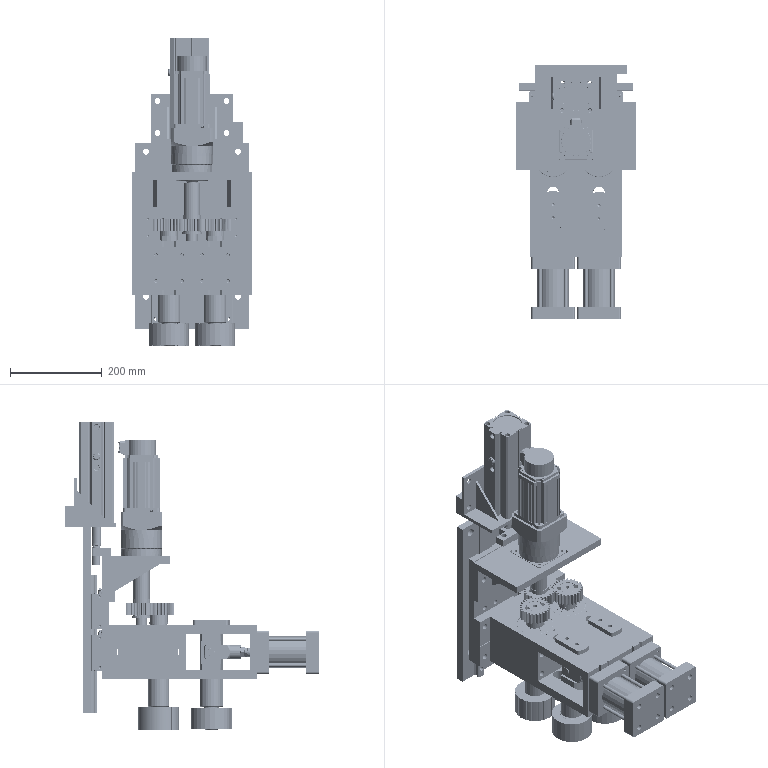Assembly | SolidWorks | mm | 89 component files | 297 solids | 8207 faces | box 260 x 553 x 669.11 mm | volume 14748799 mm3 | plane 3298 | cylinder 2702 | sphere 920 | cone 754 | torus 297 | spline 236 | commonest cylinder face diameters 0.4 x322 10.8 x192 39.85 x160 37.15 x160 4.6 x88 5 x78 67.5 x75 56.25 x75
Bill of materials:
NewCurveBender6203Bearing-DoubleWheel | 1 |  | Thick annular ring with a plain central bore and rounded outer and inner edges.
NewCurveBender6205RZBearing-DoubleWheel | 4 |  | Short, thick annular ring with a plain through bore, a cylindrical outer face and small edge rounds. Each face shows concentric steps or grooves between the inner and outer rims, so the ring looks like it is built from separate inner and outer rings with a recessed band between them.
NewCurveBender6208RSBearing-DoubleWheel | 4 |  | Plain flat annular ring (washer- or spacer-like) with a central through bore. The ring is wide and the part is thin compared with its diameter. The edges are slightly rounded or chamfered.
NewTypeCurveBender34320001-DoubleWheel | 4 |  | Angled fitting: cylindrical shank with chamfered end, a hex collar, a domed body, and an angled branch with a second hex flat and a tapered nozzle with a small orifice.
NewTypeCurveBender920018A1-DoubleWheel | 8 |  | Flat rectangular plate with chamfered corners, a central U-shaped notch with rounded side reliefs, two small through holes and one larger round through hole.
NewTypeCurveBenderDoubleWheel | 4 |  | Cylindrical cap-like body with a thin flange at the base and a chamfered top edge to a flat top face.
NewTypeCurveBenderHG20-DoubleWheel | 16 |  | Round-head pin or screw-like part with a cross-shaped recess in a low domed head and a plain cylindrical shank with chamfered tip.
NewTypeCurveBenderHGH20CAZ0C-DoubleWheel | 4 |  | Rectangular block with a U-channel end profile (chamfered corners, rounded side reliefs), a large cone-bottomed hole and two smaller holes on the end face, cone-bottomed holes on the side faces, and shallow lengthwise grooves and steps.
NewCurveBenderHGW20GuideRail210Long-DoubleWheel | 2 |  | Long straight bar with a constant profile (chamfered top corners, angled side recesses, rounded side grooves near the base) and a row of evenly spaced counterbored through holes along its length.
NewCurveBenderLowerRebarWheelAxis-DoubleWheel | 2 | 45 | Stepped cylindrical shaft with two opposite slots at one end, a small conical centre hole in that end face, circumferential grooves, a larger diameter collar section and a smaller end stub.
NewTypeCurveBenderM16x1_5-Nut-DoubleWheel | 2 |  | Thin hexagonal nut-like part with a large plain bore and chamfered corners on both faces.
NewTypeCurveBenderM16X150Y-DoubleWheel | 2 |  | Fork-shaped clevis-like body with a hollow cylindrical boss at one end, two parallel prongs separated by a rectangular slot, and a cross pin passing through both prongs with retaining features at each end.
NewCurveBenderTelescopicMotor-DoubleWheel | 1 |  | Housing with a square cross-section and a long body. It has a square mounting flange with four corner through holes at one end and a cylindrical output shaft sticking out from a pilot boss. A larger cylindrical cap sits on the opposite end, with a small block-shaped protrusion on its side. The flat sides of the body carry long grooves or ribs.
NewCurveBenderTelescopicReducer-DoubleWheel | 1 |  | Stepped housing. It has a square input-side block with chamfered corners, then a cylindrical body, then a square flange with four corner holes, then a cylindrical pilot, and finally a protruding cylindrical output shaft. The square end face has a recessed circular pocket, a central bore with a keyway, and several through or tapped holes.
NewCurveBenderUpperRebarWheelAxis-DoubleWheel | 2 | 45 | Stepped shaft with a flattened rectangular tang at one end carrying a cross hole and side notches, two small cone-bottomed holes in the tang end face, a larger cylindrical collar, and a smaller stub with a groove near its end.
NewTypeCurveBenderCylinderPlate-DoubleWheel | 1 |  | T-shaped flat block: a rectangular base with a central tab with rounded corners on one edge, a large through hole in the tab, and two smaller through holes in the base.
NewTypeCurveBenderDoubleTelescopicCylinderBasePlate-DoubleWheel | 1 |  | L-shaped angle bracket: flat base plate and perpendicular upright plate joined by two triangular gusset ribs; base has a large central round hole with four small holes around it, upright has four holes near its corners.
NewTypeCurveBenderMotorAxis-DoubleWheel | 1 |  | Stepped cylindrical shaft or sleeve: long main cylinder with a bore and keyway notch at the top end, two circumferential grooves in a middle band, a thin flange collar near the lower end, an elongated slot in the side wall, and two smaller stepped spigots at the bottom.
NewCurveBender(New)ReducerBasePlate-DoubleWheel | 1 |  | Thin rectangular plate with two through holes near its ends, a shallow step or groove running along one long edge, and a small rectangular notch at the middle of that edge.
NewCurveBender(New)Triangle-DoubleWheel | 2 |  | Flat right-triangle plate of uniform thickness with no holes, shaped like a gusset or wedge plate.
NewTypeCurveBenderReducerPlate-DoubleWheel | 1 |  | Rectangular flat plate with a large central circular hole, four small holes in a square pattern around it, and a shallow recessed pocket around the hole on one face; one end shows a small stepped tab.
NewTypeCurveBenderReinforcement | 1 |  | Solid rectangular bar with two round through holes spaced along its length, one near each end.
NewTypeCurveBenderReinforcementActiveGearM2.5x25-DoubleWheel | 3 |  | Spur-type gear with straight external teeth (about 25-30) around a ring, a large central bore, and two rectangular keyway notches on opposite sides of the bore.
NewTypeCurveBenderReinforcementFeedingWheel-DoubleWheel | 2 | Cr12MoV | Cylindrical hub or wheel with many small shallow rectangular notches around its outer edge, and a central bore with a single keyway notch.
NewTypeCurveBenderReinforcementPressingWheel-DoubleWheel | 2 |  | Plain thick-walled cylindrical ring (bushing or spacer shape) with a central through bore; an internal edge line inside the bore suggests a step or chamfer.
NewTypeCurveBenderReinforcementSeatBase-DoubleWheel | 1 |  | Thick rectangular plate with eight through holes (two pairs near each end), a groove along one face, and a small rectangular notch at the middle of one long edge.
NewTypeCurveBenderReinforcementSeatBasePlate-DoubleWheel | 1 | Q235 | Nearly square flat plate with multiple hole patterns: six larger holes along the two side edges, sixteen smaller holes in four 2x2 groups, a groove across one face, shallow stepped recesses and a central notch along one edge, and two holes drilled into that edge.
NewTypeCurveBenderReinforcementSeatUpperWheelBox1-DoubleWheel | 1 |  | Flat rectangular plate with two large circular through holes, each surrounded by four small holes in a square pattern, and four rectangular tabs sticking out from the long edges (two per side, lined up with the large holes).
NewTypeCurveBenderReinforcementSeatUpperWheelBox2-DoubleWheel | 1 |  | Flat rectangular plate with four through holes near the corners and two pairs of rectangular tabs sticking out of opposite long edges.
NewTypeCurveBenderReinforcementSeatUpperWheelBox3-DoubleWheel | 2 |  | Flat, nearly square plate with two parallel elongated slots and four rectangular edge notches with chamfered entry corners.
NewTypeCurveBenderReinforcementSeatUpperWheelBox4-DoubleWheel | 1 |  | Rectangular block with two large stepped bores and one smaller stepped bore from the top face, small holes on the side faces, and a seam or groove line around the middle of its height.
NewTypeCurveBenderReinforcementSlideRailBasePlate-DoubleWheel | 1 | Q235 | Thin rectangular plate with four larger corner holes, two rows of small holes, and shallow lengthwise grooves on both faces.
NewTypeCurveBenderReinforcementWheelStopCover-DoubleWheel | 2 |  | Thick oblong plate or bar with two round through holes along its centerline; the short ends are shallow convex arcs with rounded corners.
Mates:
1. coincident | NewTypeCurveBenderReinforcementSeatUpperWheelBox4-DoubleWheel-1 plane at (0, 0, 0) dir (0, 0, 1) | assembly plane at (0, 0, 0) dir (0, 0, 1)
2. coincident | NewTypeCurveBenderReinforcementSeatUpperWheelBox4-DoubleWheel-1 plane at (0, 0, 0) dir (-1, 0, 0) | assembly plane at (0, 0, 0) dir (1, 0, 0)
3. coincident | NewTypeCurveBenderReinforcementSeatUpperWheelBox4-DoubleWheel-1 plane at (0, 0, 0) dir (0, -1, 0) | assembly plane at (0, 0, 0) dir (0, 1, 0)
4. coincident | NewTypeCurveBenderReinforcementSeatUpperWheelBox4-DoubleWheel-1 face at (0, -133, 0) dir (0, -1, 0) | NewTypeCurveBenderReinforcementSeatUpperWheelBox2-DoubleWheel-1 face at (0, -133, 0) dir (0, 1, 0)
5. concentric | NewTypeCurveBenderReinforcementSeatUpperWheelBox4-DoubleWheel-1 face at (87.5, -133, -25) dir (0, -1, 0) r 5.1 | NewTypeCurveBenderReinforcementSeatUpperWheelBox2-DoubleWheel-1 face at (87.5, -117, -25) dir (0, -1, 0) r 6.5
6. concentric | NewTypeCurveBenderReinforcementSeatUpperWheelBox4-DoubleWheel-1 face at (87.5, -133, 25) dir (0, -1, 0) r 5.1 | NewTypeCurveBenderReinforcementSeatUpperWheelBox2-DoubleWheel-1 face at (87.5, -117, 25) dir (0, -1, 0) r 6.5
7. coincident | NewTypeCurveBenderReinforcementSeatUpperWheelBox4-DoubleWheel-1 face at (100, -133, -59) dir (1, 0, 0) | NewTypeCurveBenderReinforcementSeatUpperWheelBox3-DoubleWheel-2 face at (100, -301, -39) dir (1, 0, 0)
8. coincident | NewTypeCurveBenderReinforcementSeatUpperWheelBox4-DoubleWheel-1 face at (100, -133, -59) dir (0, 0, -1) | NewTypeCurveBenderReinforcementSeatUpperWheelBox3-DoubleWheel-2 face at (0, -217, -59) dir (0, 0, -1)
9. coincident | NewTypeCurveBenderReinforcementSeatUpperWheelBox4-DoubleWheel-1 face at (0, -133, 0) dir (0, -1, 0) | NewTypeCurveBenderReinforcementSeatUpperWheelBox3-DoubleWheel-2 face at (100, -133, -39) dir (0, 1, 0)
10. coincident | NewTypeCurveBenderReinforcementSeatUpperWheelBox4-DoubleWheel-1 face at (100, -133, -59) dir (1, 0, 0) | NewTypeCurveBenderReinforcementSeatUpperWheelBox3-DoubleWheel-1 face at (100, -301, 59) dir (1, 0, 0)
11. coincident | NewTypeCurveBenderReinforcementSeatUpperWheelBox4-DoubleWheel-1 face at (0, -133, 0) dir (0, -1, 0) | NewTypeCurveBenderReinforcementSeatUpperWheelBox3-DoubleWheel-1 face at (100, -133, 59) dir (0, 1, 0)
12. coincident | NewTypeCurveBenderReinforcementSeatUpperWheelBox4-DoubleWheel-1 face at (100, -133, 59) dir (0, 0, 1) | NewTypeCurveBenderReinforcementSeatUpperWheelBox3-DoubleWheel-1 face at (0, -217, 59) dir (0, 0, 1)
13. coincident | NewTypeCurveBenderReinforcementSeatUpperWheelBox3-DoubleWheel-2 face at (100, -301, -39) dir (0, -1, 0) | NewTypeCurveBenderReinforcementSeatUpperWheelBox1-DoubleWheel-1 face at (0, -301, 0) dir (0, -1, 0)
14. coincident | NewTypeCurveBenderReinforcementSeatUpperWheelBox3-DoubleWheel-2 face at (100, -301, -39) dir (1, 0, 0) | NewTypeCurveBenderReinforcementSeatUpperWheelBox1-DoubleWheel-1 face at (100, -301, -39) dir (1, 0, 0)
15. coincident | NewTypeCurveBenderReinforcementSeatUpperWheelBox3-DoubleWheel-1 face at (0, -217, 59) dir (0, 0, 1) | NewTypeCurveBenderReinforcementSeatUpperWheelBox1-DoubleWheel-1 face at (60, -258.716, 59) dir (0, 0, 1)
16. concentric | NewCurveBenderLowerRebarWheelAxis-DoubleWheel-1 face at (50, -88, -504.313) dir (0, 0, -1) r 22.5 | NewCurveBender6208RSBearing-DoubleWheel-1 face at (50, -88, -50) dir (0, 0, 1) r 40
17. concentric | NewCurveBenderLowerRebarWheelAxis-DoubleWheel-2 face at (-50, -88, -504.313) dir (0, 0, -1) r 19.75 | NewCurveBender6208RSBearing-DoubleWheel-4 face at (-50, -88, 50) dir (0, 0, 1) r 40
18. concentric | NewCurveBenderLowerRebarWheelAxis-DoubleWheel-1 face at (50, -88, -504.313) dir (0, 0, -1) r 19.75 | NewCurveBender6208RSBearing-DoubleWheel-2 face at (50, -88, 50) dir (0, 0, 1) r 40
19. coincident | NewCurveBenderLowerRebarWheelAxis-DoubleWheel-2 face at (-57.753, -106.436, 59) dir (0, 0, 1) | NewCurveBender6208RSBearing-DoubleWheel-4 face at (-11.557, -82.057, 59) dir (0, 0, 1)
20. coincident | NewCurveBenderLowerRebarWheelAxis-DoubleWheel-1 face at (61.035, -71.32, 59) dir (0, 0, 1) | NewCurveBender6208RSBearing-DoubleWheel-2 face at (88.443, -82.057, 59) dir (0, 0, 1)
21. coincident | NewCurveBenderLowerRebarWheelAxis-DoubleWheel-1 face at (68.765, -100.415, -59) dir (0, 0, 1) | NewCurveBender6208RSBearing-DoubleWheel-1 face at (77.177, -83.798, -59) dir (0, 0, -1)
22. coincident | NewCurveBenderLowerRebarWheelAxis-DoubleWheel-2 face at (-70.741, -79.278, -59) dir (0, 0, 1) | NewCurveBender6208RSBearing-DoubleWheel-3 face at (-22.823, -83.798, -59) dir (0, 0, -1)
23. concentric | NewCurveBenderLowerRebarWheelAxis-DoubleWheel-1 face at (50, -88, -504.313) dir (0, 0, -1) r 22.5 | NewTypeCurveBenderReinforcementFeedingWheel-DoubleWheel-1 face at (50, -88, -169) dir (0, 0, 1) r 17.5
24. coincident | NewCurveBenderLowerRebarWheelAxis-DoubleWheel-1 face at (64.595, -97.656, -119) dir (0, 0, -1) | NewTypeCurveBenderReinforcementFeedingWheel-DoubleWheel-1 face at (50, -88, -119) dir (0, 0, 1)
25. concentric | NewCurveBenderLowerRebarWheelAxis-DoubleWheel-2 face at (-50, -88, -504.313) dir (0, 0, -1) r 22.5 | NewTypeCurveBenderReinforcementFeedingWheel-DoubleWheel-2 face at (-50, -88, -169) dir (0, 0, 1) r 17.5
26. coincident | NewCurveBenderLowerRebarWheelAxis-DoubleWheel-2 face at (-66.132, -81.216, -119) dir (0, 0, -1) | NewTypeCurveBenderReinforcementFeedingWheel-DoubleWheel-2 face at (-50, -88, -119) dir (0, 0, 1)
27. coincident | NewCurveBenderLowerRebarWheelAxis-DoubleWheel-2 face at (-40.416, -97.455, -153) dir (0.3877, 0.9218, 0) | NewTypeCurveBenderReinforcementFeedingWheel-DoubleWheel-2 face at (-32.765, -100.672, -169) dir (0.3877, 0.9218, 0)
28. coincident | NewCurveBenderLowerRebarWheelAxis-DoubleWheel-1 face at (42.334, -76.933, -153) dir (-0.5518, -0.834, 0) | NewTypeCurveBenderReinforcementFeedingWheel-DoubleWheel-1 face at (35.412, -72.353, -169) dir (-0.5518, -0.834, 0)
29. concentric | NewTypeCurveBenderReinforcementSeatUpperWheelBox4-DoubleWheel-1 face at (50, -88, -41) dir (0, 0, -1) r 40 | NewCurveBenderLowerRebarWheelAxis-DoubleWheel-1 face at (50, -88, -504.313) dir (0, 0, -1) r 22.5
30. coincident | NewTypeCurveBenderReinforcementSeatUpperWheelBox4-DoubleWheel-1 face at (100, -133, -59) dir (0, 0, -1) | NewCurveBender6208RSBearing-DoubleWheel-1 face at (77.177, -83.798, -59) dir (0, 0, -1)
31. concentric | NewTypeCurveBenderReinforcementSeatUpperWheelBox4-DoubleWheel-1 face at (-50, -88, -41) dir (0, 0, -1) r 40 | NewCurveBenderLowerRebarWheelAxis-DoubleWheel-2 face at (-50, -88, -504.313) dir (0, 0, -1) r 22.5
32. coincident | NewTypeCurveBenderReinforcementSeatUpperWheelBox3-DoubleWheel-2 face at (0, -217, -59) dir (0, 0, -1) | NewCurveBender6208RSBearing-DoubleWheel-3 face at (-11.557, -82.057, -59) dir (0, 0, -1)
33. concentric | NewCurveBenderLowerRebarWheelAxis-DoubleWheel-1 face at (50, -88, -504.313) dir (0, 0, -1) r 19 | NewTypeCurveBenderReinforcementActiveGearM2.5x25-DoubleWheel-1 face at (50, -88, 106) dir (0, 0, -1) r 19
34. coincident | NewCurveBenderLowerRebarWheelAxis-DoubleWheel-1 face at (65.846, -98.484, 106) dir (0, 0, 1) | NewTypeCurveBenderReinforcementActiveGearM2.5x25-DoubleWheel-1 face at (50, -88, 106) dir (0, 0, 1)
35. coincident | NewCurveBenderLowerRebarWheelAxis-DoubleWheel-1 face at (64.435, -91.555, 106) dir (-0.5518, -0.834, 0) | NewTypeCurveBenderReinforcementActiveGearM2.5x25-DoubleWheel-1 face at (33.786, -71.277, 106) dir (-0.5518, -0.834, 0)
36. concentric | NewCurveBenderLowerRebarWheelAxis-DoubleWheel-2 face at (-50, -88, -504.313) dir (0, 0, -1) r 19 | NewTypeCurveBenderReinforcementActiveGearM2.5x25-DoubleWheel-2 face at (-50, -88, 106) dir (0, 0, -1) r 19
37. coincident | NewCurveBenderLowerRebarWheelAxis-DoubleWheel-2 face at (-64.844, -87.182, 106) dir (0.3877, 0.9218, 0) | NewTypeCurveBenderReinforcementActiveGearM2.5x25-DoubleWheel-2 face at (-30.967, -101.428, 106) dir (0.3877, 0.9218, 0)
38. coincident | NewCurveBenderLowerRebarWheelAxis-DoubleWheel-2 face at (-67.514, -80.634, 106) dir (0, 0, 1) | NewTypeCurveBenderReinforcementActiveGearM2.5x25-DoubleWheel-2 face at (-50, -88, 106) dir (0, 0, 1)
39. coincident | NewTypeCurveBenderReinforcementSeatUpperWheelBox1-DoubleWheel-1 face at (0, -301, 0) dir (0, -1, 0) | NewCurveBenderSC63x40Cylinder-DoubleWheel-1/NewTypeCurveBenderSC-63x40(0)_c-DoubleWheel-1 face at (7.387, -301, 42.613) dir (0, 1, 0)
40. concentric | NewTypeCurveBenderReinforcementSeatUpperWheelBox1-DoubleWheel-1 face at (-50, -287, 0) dir (0, -1, 0) r 25 | NewCurveBenderSC63x40Cylinder-DoubleWheel-2/NewTypeCurveBenderSC-63x40(0)_c-DoubleWheel-1 face at (-50, -301, 0) dir (0, 1, 0) r 19
41. coincident | NewTypeCurveBenderReinforcementSeatUpperWheelBox1-DoubleWheel-1 face at (0, -301, 0) dir (0, -1, 0) | NewCurveBenderSC63x40Cylinder-DoubleWheel-2/NewTypeCurveBenderSC-63x40(0)_c-DoubleWheel-1 face at (-92.613, -301, 42.613) dir (0, 1, 0)
42. perpendicular | NewCurveBenderSC63x40Cylinder-DoubleWheel-1/NewTypeCurveBenderSC-63x40(0)_c-DoubleWheel-1 face at (7.387, -328.5, -47) dir (0, 0, -1) | NewCurveBenderSC63x40Cylinder-DoubleWheel-2/NewTypeCurveBenderSC-63x40(0)_c-DoubleWheel-1 face at (-97, -328.5, 42.613) dir (-1, 0, 0)
43. coincident | NewTypeCurveBenderReinforcementSeatUpperWheelBox3-DoubleWheel-1 face at (0, -217, 59) dir (0, 0, 1) | NewCurveBenderUpperRebarWheelAxis-DoubleWheel-2 face at (50, -204, 59) dir (0, 0, 1)
44. coincident | NewTypeCurveBenderReinforcementSeatUpperWheelBox3-DoubleWheel-1 face at (63, -226, 39) dir (-1, 0, 0) | NewCurveBenderUpperRebarWheelAxis-DoubleWheel-2 face at (63, -183.826, -59) dir (1, 0, 0)
45. concentric | NewCurveBenderUpperRebarWheelAxis-DoubleWheel-2 face at (25.25, -204, 0) dir (1, 0, 0) r 8.1 | NewCurveBenderSC63x40Cylinder-DoubleWheel-1/NewTypeCurveBenderM16X150Y-DoubleWheel-2 face at (69.5, -204, 0) dir (-1, 0, 0) r 8
46. width | NewCurveBenderSC63x40Cylinder-DoubleWheel-1/NewTypeCurveBenderM16X150Y-DoubleWheel-2 face at (66, -190.075, -48) dir (1, 0, 0) | NewCurveBenderSC63x40Cylinder-DoubleWheel-1/NewTypeCurveBenderM16X150Y-DoubleWheel-2 face at (34, -246, -48) dir (-1, 0, 0) | NewCurveBenderUpperRebarWheelAxis-DoubleWheel-2 face at (42, -228.75, 25) dir (-1, 0, 0) | NewCurveBenderUpperRebarWheelAxis-DoubleWheel-2 face at (58, -228.75, 25) dir (1, 0, 0)
47. coincident | NewTypeCurveBenderReinforcementSeatUpperWheelBox3-DoubleWheel-1 face at (0, -217, 59) dir (0, 0, 1) | NewCurveBenderUpperRebarWheelAxis-DoubleWheel-1 face at (-50, -201.632, 59) dir (0, 0, 1)
48. concentric | NewCurveBenderUpperRebarWheelAxis-DoubleWheel-1 face at (-74.75, -201.632, 0) dir (1, 0, 0) r 8.1 | NewCurveBenderSC63x40Cylinder-DoubleWheel-2/NewTypeCurveBenderM16X150Y-DoubleWheel-2 face at (-69.5, -201.632, 0) dir (1, 0, 0) r 8
49. width | NewCurveBenderSC63x40Cylinder-DoubleWheel-2/NewTypeCurveBenderM16X150Y-DoubleWheel-2 face at (-66, -187.707, 48) dir (-1, 0, 0) | NewCurveBenderSC63x40Cylinder-DoubleWheel-2/NewTypeCurveBenderM16X150Y-DoubleWheel-2 face at (-34, -243.632, 48) dir (1, 0, 0) | NewCurveBenderUpperRebarWheelAxis-DoubleWheel-1 face at (-42, -226.382, 25) dir (1, 0, 0) | NewCurveBenderUpperRebarWheelAxis-DoubleWheel-1 face at (-58, -226.382, 25) dir (-1, 0, 0)
50. concentric | NewCurveBenderUpperRebarWheelAxis-DoubleWheel-2 face at (50, -204, 59) dir (0, 0, -1) r 12.5 | NewCurveBender6205RZBearing-DoubleWheel-1 face at (50, -204, -125) dir (0, 0, 1) r 26
51. concentric | NewCurveBenderUpperRebarWheelAxis-DoubleWheel-1 face at (-50, -201.632, 59) dir (0, 0, -1) r 12.5 | NewCurveBender6205RZBearing-DoubleWheel-8 face at (-50, -201.632, -125) dir (0, 0, 1) r 26
52. concentric | NewCurveBenderUpperRebarWheelAxis-DoubleWheel-2 face at (50, -204, 59) dir (0, 0, -1) r 12.5 | NewCurveBender6205RZBearing-DoubleWheel-2 face at (50, -204, -153) dir (0, 0, 1) r 26
53. concentric | NewCurveBenderUpperRebarWheelAxis-DoubleWheel-1 face at (-50, -201.632, 59) dir (0, 0, -1) r 12.5 | NewCurveBender6205RZBearing-DoubleWheel-7 face at (-50, -201.632, -153) dir (0, 0, 1) r 26
54. distance | NewCurveBenderUpperRebarWheelAxis-DoubleWheel-1 face at (-62.5, -201.632, -169) dir (0, 0, -1) | NewCurveBender6205RZBearing-DoubleWheel-7 face at (-44.617, -177.218, -164) dir (0, 0, -1)
55. coincident | NewCurveBender6205RZBearing-DoubleWheel-2 face at (49.19, -179.013, -164) dir (0, 0, -1) | NewCurveBender6205RZBearing-DoubleWheel-7 face at (-44.617, -177.218, -164) dir (0, 0, -1)
56. concentric | NewCurveBenderUpperRebarWheelAxis-DoubleWheel-1 face at (-50, -201.632, 59) dir (0, 0, -1) r 24.75 | NewTypeCurveBenderReinforcementPressingWheel-DoubleWheel-1 face at (-50, -201.632, -121) dir (0, 0, -1) r 44
57. coincident | NewCurveBender6205RZBearing-DoubleWheel-8 face at (-50, -176.632, -121) dir (0, 0, 1) | NewTypeCurveBenderReinforcementPressingWheel-DoubleWheel-1 face at (-50, -201.632, -121) dir (0, 0, 1)
58. concentric | NewCurveBenderUpperRebarWheelAxis-DoubleWheel-2 face at (50, -204, 59) dir (0, 0, -1) r 24.75 | NewTypeCurveBenderReinforcementPressingWheel-DoubleWheel-2 face at (50, -204, -121) dir (0, 0, -1) r 44
59. coincident | NewCurveBender6205RZBearing-DoubleWheel-1 face at (50, -179, -121) dir (0, 0, 1) | NewTypeCurveBenderReinforcementPressingWheel-DoubleWheel-2 face at (50, -204, -121) dir (0, 0, 1)
60. concentric | NewTypeCurveBenderReinforcementSeatUpperWheelBox4-DoubleWheel-1 face at (0, -50.5, 47) dir (0, 0, 1) r 20 | NewTypeCurveBenderMotorAxis-DoubleWheel-1 face at (0, -50.5, 43) dir (0, 0, 1) r 18
61. coincident | NewTypeCurveBenderReinforcementSeatUpperWheelBox4-DoubleWheel-1 face at (0, -50.5, 43) dir (0, 0, 1) | NewTypeCurveBenderMotorAxis-DoubleWheel-1 face at (0, -50.5, 43) dir (0, 0, -1)
62. concentric | NewTypeCurveBenderMotorAxis-DoubleWheel-1 face at (0, -50.5, 43) dir (0, 0, 1) r 12.5 | NewCurveBender6203Bearing-DoubleWheel-1 face at (0, -50.5, 59) dir (0, 0, -1) r 20
63. coincident | NewTypeCurveBenderReinforcementSeatUpperWheelBox4-DoubleWheel-1 face at (100, -133, 59) dir (0, 0, 1) | NewCurveBender6203Bearing-DoubleWheel-1 face at (0, -50.5, 59) dir (0, 0, 1)
64. concentric | NewTypeCurveBenderMotorAxis-DoubleWheel-1 face at (0, -50.5, 43) dir (0, 0, 1) r 18 | NewTypeCurveBenderReinforcementActiveGearM2.5x25-DoubleWheel-3 face at (0, -50.5, 106) dir (0, 0, -1) r 19
65. coincident | NewTypeCurveBenderMotorAxis-DoubleWheel-1 face at (14.462, -53.944, 97.5) dir (-0.5454, -0.8382, 0) | NewTypeCurveBenderReinforcementActiveGearM2.5x25-DoubleWheel-3 face at (21.796, -58.716, 106) dir (-0.5454, -0.8382, 0)
66. coincident | NewTypeCurveBenderReinforcementActiveGearM2.5x25-DoubleWheel-1 face at (50, -88, 106) dir (0, 0, 1) | NewTypeCurveBenderReinforcementActiveGearM2.5x25-DoubleWheel-3 face at (0, -50.5, 106) dir (0, 0, 1)
67. gear | NewTypeCurveBenderReinforcementActiveGearM2.5x25-DoubleWheel-1 sketch segment at (50, -88, 93.5) dir (0, 0, -1) r 31.25 | NewTypeCurveBenderReinforcementActiveGearM2.5x25-DoubleWheel-3 sketch segment at (0, -50.5, 93.5) dir (0, 0, -1) r 31.25
68. gear | NewTypeCurveBenderReinforcementActiveGearM2.5x25-DoubleWheel-2 sketch segment at (-50, -88, 93.5) dir (0, 0, -1) r 31.25 | NewTypeCurveBenderReinforcementActiveGearM2.5x25-DoubleWheel-3 sketch segment at (0, -50.5, 93.5) dir (0, 0, -1) r 31.25
69. coincident | NewCurveBenderUpperRebarWheelAxis-DoubleWheel-2 face at (50, -204, 59) dir (0, 0, 1) | NewTypeCurveBenderReinforcementWheelStopCover-DoubleWheel-1 face at (62.5, -236.692, 59) dir (0, 0, -1)
70. concentric | NewCurveBenderUpperRebarWheelAxis-DoubleWheel-2 face at (50, -219, 59) dir (0, 0, 1) r 3.4 | NewTypeCurveBenderReinforcementWheelStopCover-DoubleWheel-1 face at (50, -219, 59) dir (0, 0, 1) r 4.5
71. concentric | NewCurveBenderUpperRebarWheelAxis-DoubleWheel-2 face at (50, -189, 59) dir (0, 0, 1) r 3.4 | NewTypeCurveBenderReinforcementWheelStopCover-DoubleWheel-1 face at (50, -189, 59) dir (0, 0, 1) r 4.5
72. coincident | NewCurveBenderUpperRebarWheelAxis-DoubleWheel-1 face at (-50, -201.632, 59) dir (0, 0, 1) | NewTypeCurveBenderReinforcementWheelStopCover-DoubleWheel-2 face at (-62.5, -234.324, 59) dir (0, 0, -1)
73. concentric | NewCurveBenderUpperRebarWheelAxis-DoubleWheel-1 face at (-50, -216.632, 59) dir (0, 0, 1) r 3.4 | NewTypeCurveBenderReinforcementWheelStopCover-DoubleWheel-2 face at (-50, -216.632, 69) dir (0, 0, -1) r 4.5
74. concentric | NewCurveBenderUpperRebarWheelAxis-DoubleWheel-1 face at (-50, -186.632, 59) dir (0, 0, 1) r 3.4 | NewTypeCurveBenderReinforcementWheelStopCover-DoubleWheel-2 face at (-50, -186.632, 69) dir (0, 0, -1) r 4.5
75. concentric | NewTypeCurveBenderMotorAxis-DoubleWheel-1 face at (0, -50.5, 145) dir (0, 0, 1) r 11 | NewCurveBenderTelescopicMotorGearbox-DoubleWheel-1/NewCurveBenderTelescopicReducer-DoubleWheel-1 face at (0, -50.5, 201) dir (0, 0, 1) r 11
76. distance | NewCurveBenderTelescopicMotorGearbox-DoubleWheel-1/NewCurveBenderTelescopicReducer-DoubleWheel-1 face at (0, -64.54, 189.5) dir (0, 0, -1) | NewTypeCurveBenderMotorAxis-DoubleWheel-1 face at (-15.087, -40.683, 185) dir (0, 0, 1)
77. coincident | NewTypeCurveBenderReinforcementSeatUpperWheelBox4-DoubleWheel-1 face at (100, -133, -59) dir (0, 0, -1) | NewTypeCurveBenderReinforcementSeatBasePlate-DoubleWheel-1 face at (-130, 20, -59) dir (0, 0, -1)
78. coincident | NewTypeCurveBenderReinforcementSeatUpperWheelBox4-DoubleWheel-1 face at (100, -133, -59) dir (0, 0, -1) | NewTypeCurveBenderReinforcementSeatBase-DoubleWheel-1 face at (130, 0, -59) dir (0, 0, -1)
79. coincident | NewTypeCurveBenderReinforcementSeatUpperWheelBox4-DoubleWheel-1 face at (0, 0, 0) dir (0, 1, 0) | NewTypeCurveBenderReinforcementSeatBase-DoubleWheel-1 face at (0, 0, 0) dir (0, -1, 0)
80. coincident | NewTypeCurveBenderReinforcementSeatBasePlate-DoubleWheel-1 face at (130, 20, -59) dir (1, 0, 0) | NewTypeCurveBenderReinforcementSeatBase-DoubleWheel-1 face at (130, 0, -59) dir (1, 0, 0)
81. coincident | NewTypeCurveBenderReinforcementSeatBasePlate-DoubleWheel-1 face at (0, 20, 0.5) dir (0, -1, 0) | NewTypeCurveBenderReinforcementSeatBase-DoubleWheel-1 face at (0, 20, 0) dir (0, 1, 0)
82. coincident | NewTypeCurveBenderReinforcementSeatBasePlate-DoubleWheel-1 face at (130, 20, -59) dir (1, 0, 0) | NewTypeCurveBenderReducerPlate-DoubleWheel-2/NewCurveBender(New)ReducerBasePlate-DoubleWheel-1 face at (130, 8, 108) dir (1, 0, 0)
83. concentric | NewTypeCurveBenderReinforcementSeatBasePlate-DoubleWheel-1 face at (110, 20, 158) dir (0, -1, 0) r 5.1 | NewTypeCurveBenderReducerPlate-DoubleWheel-2/NewCurveBender(New)ReducerBasePlate-DoubleWheel-1 face at (110, 20, 158) dir (0, -1, 0) r 6.75
84. coincident | NewTypeCurveBenderReinforcementSeatBasePlate-DoubleWheel-1 face at (0, 20, 0.5) dir (0, -1, 0) | NewTypeCurveBenderReducerPlate-DoubleWheel-2/NewCurveBender(New)ReducerBasePlate-DoubleWheel-1 face at (0, 20, 158) dir (0, 1, 0)
85. parallel | NewCurveBenderTelescopicMotorGearbox-DoubleWheel-1/NewCurveBenderTelescopicReducer-DoubleWheel-1 face at (-39.686, -95.5, 265.45) dir (0, -1, 0) | NewTypeCurveBenderReducerPlate-DoubleWheel-2/NewTypeCurveBenderReducerPlate-DoubleWheel-1 face at (130, -112, 208) dir (0, -1, 0)
86. width | NewTypeCurveBenderReinforcementSeatBase-DoubleWheel-1 face at (130, 0, -59) dir (1, 0, 0) | NewTypeCurveBenderReinforcementSeatBase-DoubleWheel-1 face at (-130, 0, -59) dir (-1, 0, 0) | NewTypeCurveBenderReinforcementSeatUpperWheelBox4-DoubleWheel-1 face at (-100, -133, -59) dir (-1, 0, 0) | NewTypeCurveBenderReinforcementSeatUpperWheelBox4-DoubleWheel-1 face at (100, -133, -59) dir (1, 0, 0)
87. concentric | NewTypeCurveBenderReinforcementSeatBasePlate-DoubleWheel-1 face at (96, 20, 70.63) dir (0, -1, 0) r 3.3 | NewCurveBenderHG20Slider-DoubleWheel-1/NewTypeCurveBenderHGH20CAZ0C-DoubleWheel-1 face at (96, 41.393, 70.63) dir (0, -1, 0) r 2.067
88. concentric | NewTypeCurveBenderReinforcementSeatBasePlate-DoubleWheel-1 face at (64, 20, 70.63) dir (0, -1, 0) r 3.3 | NewCurveBenderHG20Slider-DoubleWheel-1/NewTypeCurveBenderHGH20CAZ0C-DoubleWheel-1 face at (64, 41.393, 70.63) dir (0, -1, 0) r 2.067
89. coincident | NewTypeCurveBenderReinforcementSeatBasePlate-DoubleWheel-1 face at (102, 33, 60) dir (0, 1, 0) | NewCurveBenderHG20Slider-DoubleWheel-1/NewTypeCurveBenderHGH20CAZ0C-DoubleWheel-1 face at (84, 33, 63.38) dir (0, -1, 0)
90. concentric | NewTypeCurveBenderReinforcementSeatBasePlate-DoubleWheel-1 face at (-96, 20, 106.63) dir (0, -1, 0) r 3.3 | NewCurveBenderHG20Slider-DoubleWheel-2/NewTypeCurveBenderHGH20CAZ0C-DoubleWheel-1 face at (-96, 41.393, 106.63) dir (0, -1, 0) r 2.067
91. concentric | NewTypeCurveBenderReinforcementSeatBasePlate-DoubleWheel-1 face at (-96, 20, 70.63) dir (0, -1, 0) r 3.3 | NewCurveBenderHG20Slider-DoubleWheel-2/NewTypeCurveBenderHGH20CAZ0C-DoubleWheel-1 face at (-96, 41.393, 70.63) dir (0, -1, 0) r 2.067
92. coincident | NewTypeCurveBenderReinforcementSeatBasePlate-DoubleWheel-1 face at (-102, 33, 60) dir (0, 1, 0) | NewCurveBenderHG20Slider-DoubleWheel-2/NewTypeCurveBenderHGH20CAZ0C-DoubleWheel-1 face at (-76, 33, 63.38) dir (0, -1, 0)
93. coincident | NewCurveBenderHG20Slider-DoubleWheel-1/NewTypeCurveBenderHGH20CAZ0C-DoubleWheel-1 face at (90, 49.7, 63.38) dir (-1, 0, 0) | NewCurveBenderHGW20GuideRail210Long-DoubleWheel-1 face at (90, 48.1, 78.11) dir (1, 0, 0)
94. coincident | NewCurveBenderHG20Slider-DoubleWheel-1/NewTypeCurveBenderHGH20CAZ0C-DoubleWheel-1 face at (87.4, 45.5, 63.38) dir (0, 1, 0) | NewCurveBenderHGW20GuideRail210Long-DoubleWheel-1 face at (72.6, 45.5, 78.11) dir (0, -1, 0)
95. coincident | NewCurveBenderHG20Slider-DoubleWheel-2/NewTypeCurveBenderHGH20CAZ0C-DoubleWheel-1 face at (-70, 49.7, 63.38) dir (-1, 0, 0) | NewCurveBenderHGW20GuideRail210Long-DoubleWheel-2 face at (-70, 48.1, 78.11) dir (1, 0, 0)
96. coincident | NewCurveBenderHG20Slider-DoubleWheel-2/NewTypeCurveBenderHGH20CAZ0C-DoubleWheel-1 face at (-72.6, 45.5, 63.38) dir (0, 1, 0) | NewCurveBenderHGW20GuideRail210Long-DoubleWheel-2 face at (-87.4, 45.5, 78.11) dir (0, -1, 0)
97. coincident | NewCurveBenderHGW20GuideRail210Long-DoubleWheel-1 face at (89.8, 52.2, -131.89) dir (0, 0, -1) | NewTypeCurveBenderReinforcementSlideRailBasePlate-DoubleWheel-1 face at (-125, 60, -131.89) dir (0, 0, -1)
98. coincident | NewCurveBenderHGW20GuideRail210Long-DoubleWheel-2 face at (-70.2, 52.2, -131.89) dir (0, 0, -1) | NewTypeCurveBenderReinforcementSlideRailBasePlate-DoubleWheel-1 face at (-125, 60, -131.89) dir (0, 0, -1)
99. coincident | NewCurveBenderHGW20GuideRail210Long-DoubleWheel-1 face at (89.01, 63, 78.11) dir (0, 1, 0) | NewTypeCurveBenderReinforcementSlideRailBasePlate-DoubleWheel-1 face at (90, 63, 273.11) dir (0, -1, 0)
100. concentric | NewCurveBenderHGW20GuideRail210Long-DoubleWheel-1 face at (80, 45.5, -111.89) dir (0, 1, 0) r 4.75 | NewTypeCurveBenderReinforcementSlideRailBasePlate-DoubleWheel-1 face at (80, 60, -111.89) dir (0, -1, 0) r 2.5
101. concentric | NewTypeCurveBenderReinforcementSeatBasePlate-DoubleWheel-1 face at (-96, 20, -19.37) dir (0, -1, 0) r 3.3 | NewCurveBenderHG20Slider-DoubleWheel-3/NewTypeCurveBenderHGH20CAZ0C-DoubleWheel-1 face at (-96, 41.393, -19.37) dir (0, -1, 0) r 2.067
102. concentric | NewTypeCurveBenderReinforcementSeatBasePlate-DoubleWheel-1 face at (-64, 20, -19.37) dir (0, -1, 0) r 3.3 | NewCurveBenderHG20Slider-DoubleWheel-3/NewTypeCurveBenderHGH20CAZ0C-DoubleWheel-1 face at (-64, 41.393, -19.37) dir (0, -1, 0) r 2.067
103. coincident | NewTypeCurveBenderReinforcementSeatBasePlate-DoubleWheel-1 face at (-102, 33, 60) dir (0, 1, 0) | NewCurveBenderHG20Slider-DoubleWheel-3/NewTypeCurveBenderHGH20CAZ0C-DoubleWheel-1 face at (-76, 33, -26.62) dir (0, -1, 0)
104. concentric | NewTypeCurveBenderReinforcementSeatBasePlate-DoubleWheel-1 face at (96, 20, -19.37) dir (0, -1, 0) r 3.3 | NewCurveBenderHG20Slider-DoubleWheel-4/NewTypeCurveBenderHGH20CAZ0C-DoubleWheel-1 face at (96, 41.393, -19.37) dir (0, -1, 0) r 2.067
105. concentric | NewTypeCurveBenderReinforcementSeatBasePlate-DoubleWheel-1 face at (64, 20, -19.37) dir (0, -1, 0) r 3.3 | NewCurveBenderHG20Slider-DoubleWheel-4/NewTypeCurveBenderHGH20CAZ0C-DoubleWheel-1 face at (64, 41.393, -19.37) dir (0, -1, 0) r 2.067
106. distance | NewTypeCurveBenderCylinderPlate-DoubleWheel-1 face at (45, 15, 226) dir (0, -1, 0) | NewTypeCurveBenderReinforcementSeatBasePlate-DoubleWheel-1 face at (0, 20, 0.5) dir (0, -1, 0)
107. distance | NewTypeCurveBenderCylinderPlate-DoubleWheel-1 face at (45, 15, 226) dir (1, 0, 0) | NewTypeCurveBenderReducerPlate-DoubleWheel-2/NewCurveBender(New)ReducerBasePlate-DoubleWheel-1 face at (130, 8, 108) dir (1, 0, 0)
108. coincident | NewTypeCurveBenderReinforcementSeatBasePlate-DoubleWheel-1 face at (0, 36, 210) dir (0, 0, 1) | NewTypeCurveBenderCylinderPlate-DoubleWheel-1 face at (0, 36.5, 210) dir (0, 0, -1)
109. concentric | NewTypeCurveBenderCylinderPlate-DoubleWheel-1 face at (0, 47, 210) dir (0, 0, 1) r 10 | NewCurveBenderSDAT63x45x45Cylinder-DoubleWheel-1/NewTypeCurveBenderSDATS-63x45x45-B_4545r-DoubleWheel-1 face at (0, 47, 359.459) dir (0, 0, -1) r 10
110. distance | NewTypeCurveBenderReinforcementSlideRailBasePlate-DoubleWheel-1 face at (-125, 60, -131.89) dir (0, 0, -1) | NewTypeCurveBenderReinforcementSeatBase-DoubleWheel-1 face at (130, 0, -59) dir (0, 0, -1)
111. concentric | NewCurveBenderSDAT63x45x45Cylinder-DoubleWheel-1/NewTypeCurveBenderSDATS-63x45x45-B_4545r-DoubleWheel-1 face at (0, 47, 359.459) dir (0, 0, -1) r 10 | NewTypeCurveBenderDoubleTelescopicCylinderBasePlate-DoubleWheel-2 face at (0, 47, 283.11) dir (0, 0, -1) r 20
112. coincident | NewTypeCurveBenderReinforcementSlideRailBasePlate-DoubleWheel-1 face at (-125, 60, 273.11) dir (0, 0, 1) | NewTypeCurveBenderDoubleTelescopicCylinderBasePlate-DoubleWheel-2 face at (0, 50.5, 273.11) dir (0, 0, -1)
113. parallel | NewCurveBenderSDAT63x45x45Cylinder-DoubleWheel-1/NewTypeCurveBenderSDATS-63x45x45_4545b-DoubleWheel-1 face at (37.5, 55.4, 500.11) dir (1, 0, 0) | NewTypeCurveBenderDoubleTelescopicCylinderBasePlate-DoubleWheel-2 face at (90, 4, 273.11) dir (1, 0, 0)
114. parallel | NewTypeCurveBenderReinforcementSlideRailBasePlate-DoubleWheel-1 face at (125, 60, 273.11) dir (1, 0, 0) | NewTypeCurveBenderDoubleTelescopicCylinderBasePlate-DoubleWheel-2 face at (90, 4, 273.11) dir (1, 0, 0)
115. coincident | NewCurveBenderSDAT63x45x45Cylinder-DoubleWheel-1/NewTypeCurveBenderSDATS-63x45x45_4545b-DoubleWheel-1 face at (-0.8, 9.7, 281.11) dir (0, 0, -1) | NewTypeCurveBenderDoubleTelescopicCylinderBasePlate-DoubleWheel-2 face at (0, 50.5, 281.11) dir (0, 0, 1)
116. coincident | NewTypeCurveBenderDoubleTelescopicCylinderBasePlate-DoubleWheel-2 face at (0, 50.5, 273.11) dir (0, 0, -1) | NewTypeCurveBenderReinforcement-1 face at (110, 96, 273.11) dir (0, 0, -1)
117. parallel | NewTypeCurveBenderDoubleTelescopicCylinderBasePlate-DoubleWheel-2 face at (90, 4, 273.11) dir (1, 0, 0) | NewTypeCurveBenderReinforcement-1 face at (110, 96, 318.11) dir (1, 0, 0)
118. coincident | NewTypeCurveBenderDoubleTelescopicCylinderBasePlate-DoubleWheel-2 face at (90, 96, 378.11) dir (0, 1, 0) | NewTypeCurveBenderReinforcement-1 face at (110, 96, 318.11) dir (0, -1, 0)
119. coincident | NewTypeCurveBenderDoubleTelescopicCylinderBasePlate-DoubleWheel-2 face at (-90, 4, 273.11) dir (-1, 0, 0) | NewTypeCurveBenderReinforcement-1 face at (-90, 96, 318.11) dir (-1, 0, 0)
120. slot | NewCurveBenderUpperRebarWheelAxis-DoubleWheel-2 face at (50, -204, 59) dir (0, 0, -1) r 24 | NewTypeCurveBenderReinforcementSeatUpperWheelBox3-DoubleWheel-2 face at (37, -226, -59) dir (1, 0, 0)
121. slot | NewCurveBenderUpperRebarWheelAxis-DoubleWheel-1 face at (-50, -201.632, 59) dir (0, 0, -1) r 24 | NewTypeCurveBenderReinforcementSeatUpperWheelBox3-DoubleWheel-2 face at (-63, -226, -59) dir (1, 0, 0)
122. coincident | NewCurveBenderUpperRebarWheelAxis-DoubleWheel-2 face at (35, -204, -121) dir (0, 0, -1) | NewCurveBender6205RZBearing-DoubleWheel-1 face at (50, -190.5, -121) dir (0, 0, 1)
123. coincident | NewCurveBenderUpperRebarWheelAxis-DoubleWheel-1 face at (-65, -201.632, -121) dir (0, 0, -1) | NewCurveBender6205RZBearing-DoubleWheel-8 face at (-50, -188.132, -121) dir (0, 0, 1)
124. coincident | NewTypeCurveBenderReinforcementSeatBasePlate-DoubleWheel-1 face at (102, 33, 60) dir (0, 1, 0) | NewCurveBenderHG20Slider-DoubleWheel-4/NewTypeCurveBenderHGH20CAZ0C-DoubleWheel-1 face at (84, 33, -26.62) dir (0, -1, 0)
125. concentric | NewTypeCurveBender920018A1-DoubleWheel-1 face at (26.105, 11.307, 9.764) dir (-1, 0, 0) r 1.3 | NewTypeCurveBenderHG20-DoubleWheel-4 face at (19.365, 11.307, 9.764) dir (1, 0, 0) r 1.3
126. coincident | NewTypeCurveBender920018A1-DoubleWheel-1 face at (30.365, 11.307, 9.764) dir (1, 0, 0) | NewTypeCurveBenderHG20-DoubleWheel-4 face at (30.365, 8.557, 9.764) dir (-1, 0, 0)
127. concentric | NewTypeCurveBender920018A1-DoubleWheel-1 face at (26.105, 11.307, -22.628) dir (-1, 0, 0) r 1.3 | NewTypeCurveBenderHG20-DoubleWheel-3 face at (19.365, 11.307, -22.628) dir (1, 0, 0) r 1.3
128. coincident | NewTypeCurveBender920018A1-DoubleWheel-1 face at (30.365, 11.307, -22.628) dir (1, 0, 0) | NewTypeCurveBenderHG20-DoubleWheel-3 face at (30.365, 8.557, -22.628) dir (-1, 0, 0)
129. concentric | NewTypeCurveBender920018A1-DoubleWheel-1 face at (27.605, 21.522, -6.432) dir (-1, 0, 0) r 3.6 | NewTypeCurveBenderDoubleWheel-1 face at (28.105, 21.522, -6.432) dir (-1, 0, 0) r 3
130. concentric | NewTypeCurveBenderHGH20CAZ0C-DoubleWheel-1 face at (27.605, 11.307, -22.628) dir (-1, 0, 0) r 1.301 | NewTypeCurveBenderHG20-DoubleWheel-3 face at (19.365, 11.307, -22.628) dir (1, 0, 0) r 1.3
131. concentric | NewTypeCurveBenderHGH20CAZ0C-DoubleWheel-1 face at (27.605, 11.307, 9.764) dir (-1, 0, 0) r 1.301 | NewTypeCurveBenderHG20-DoubleWheel-4 face at (19.365, 11.307, 9.764) dir (1, 0, 0) r 1.3
132. coincident | NewTypeCurveBenderHGH20CAZ0C-DoubleWheel-1 face at (27.605, 2.122, -6.432) dir (1, 0, 0) | NewTypeCurveBender920018A1-DoubleWheel-1 face at (27.605, 2.122, -6.432) dir (-1, 0, 0)
133. coincident | NewTypeCurveBenderHGH20CAZ0C-DoubleWheel-1 face at (27.605, 2.122, -6.432) dir (1, 0, 0) | NewTypeCurveBenderDoubleWheel-1 face at (27.605, 21.522, -3.432) dir (-1, 0, 0)
134. concentric | NewTypeCurveBender920018A1-DoubleWheel-2 face at (-42.395, 11.307, -22.628) dir (1, 0, 0) r 1.3 | NewTypeCurveBenderHG20-DoubleWheel-2 face at (-35.655, 11.307, -22.628) dir (-1, 0, 0) r 1.3
135. coincident | NewTypeCurveBender920018A1-DoubleWheel-2 face at (-46.655, 11.307, -22.628) dir (-1, 0, 0) | NewTypeCurveBenderHG20-DoubleWheel-2 face at (-46.655, 14.057, -22.628) dir (1, 0, 0)
136. concentric | NewTypeCurveBender920018A1-DoubleWheel-2 face at (-42.395, 11.307, 9.764) dir (1, 0, 0) r 1.3 | NewTypeCurveBenderHG20-DoubleWheel-1 face at (-35.655, 11.307, 9.764) dir (-1, 0, 0) r 1.3
137. coincident | NewTypeCurveBender920018A1-DoubleWheel-2 face at (-46.655, 11.307, 9.764) dir (-1, 0, 0) | NewTypeCurveBenderHG20-DoubleWheel-1 face at (-46.655, 14.057, 9.764) dir (1, 0, 0)
138. concentric | NewTypeCurveBenderHGH20CAZ0C-DoubleWheel-1 face at (-33.285, 11.307, -22.628) dir (-1, 0, 0) r 1.301 | NewTypeCurveBenderHG20-DoubleWheel-2 face at (-35.655, 11.307, -22.628) dir (-1, 0, 0) r 1.3
139. concentric | NewTypeCurveBenderHGH20CAZ0C-DoubleWheel-1 face at (-33.285, 11.307, 9.764) dir (-1, 0, 0) r 1.301 | NewTypeCurveBenderHG20-DoubleWheel-1 face at (-35.655, 11.307, 9.764) dir (-1, 0, 0) r 1.3
140. coincident | NewTypeCurveBenderHGH20CAZ0C-DoubleWheel-1 face at (-43.895, 2.122, -6.432) dir (-1, 0, 0) | NewTypeCurveBender920018A1-DoubleWheel-2 face at (-43.895, 2.122, -6.432) dir (1, 0, 0)
141. concentric | NewTypeCurveBenderHGH20CAZ0C-DoubleWheel-1 face at (-33.895, 21.522, -6.432) dir (-1, 0, 0) r 3.001 | NewTypeCurveBender34320001-DoubleWheel-1 face at (-57.275, 21.522, -6.432) dir (1, 0, 0) r 3
142. coincident | NewTypeCurveBender920018A1-DoubleWheel-2 face at (-46.775, 7.615, 4.075) dir (-1, 0, 0) | NewTypeCurveBender34320001-DoubleWheel-1 face at (-46.775, 21.522, -3.432) dir (1, 0, 0)
143. coincident | NewTypeCurveBenderSC-63x40(0)_c-DoubleWheel-1 axis at (-80.9, 0, 0) dir (1, 0, 0) | NewTypeCurveBenderSC-63x40(0)_r-DoubleWheel-1 axis at (80.9, 0, 0) dir (-1, 0, 0)
144. angle | NewTypeCurveBenderSC-63x40(0)_r-DoubleWheel-1 plane at (0, 0, 0) dir (0, 0, -1) | NewTypeCurveBenderSC-63x40(0)_c-DoubleWheel-1 plane at (0, 0, 0) dir (0, 0, -1)
145. distance | NewTypeCurveBenderM16X150Y-DoubleWheel-2 face at (-33, 0, 0) dir (1, 0, 0) | NewTypeCurveBenderSC-63x40(0)_r-DoubleWheel-1 face at (-57, 0, 0) dir (-1, 0, 0)
146. distance | NewTypeCurveBenderSC-63x40(0)_r-DoubleWheel-1 face at (104, 31.25, 0) dir (1, 0, 0) | NewTypeCurveBenderSC-63x40(0)_c-DoubleWheel-1 face at (104, 31.5, 0) dir (-1, 0, 0)
147. concentric | NewTypeCurveBenderSC-63x40(0)_r-DoubleWheel-1 face at (104, 0, 0) dir (-1, 0, 0) r 8 | NewTypeCurveBenderM16x1_5-Nut-DoubleWheel-2 face at (-33, 0, 0) dir (1, 0, 0) r 8
148. concentric | NewTypeCurveBenderSC-63x40(0)_r-DoubleWheel-1 face at (104, 0, 0) dir (-1, 0, 0) r 8 | NewTypeCurveBenderM16x1_5-Nut-DoubleWheel-2 face at (-33, 0, 0) dir (1, 0, 0) r 8
149. coincident | NewTypeCurveBenderSC-63x40(0)_r-DoubleWheel-1 edge at (-25, 0, 0) dir (-1, 0, 0) r 8 | NewTypeCurveBenderM16x1_5-Nut-DoubleWheel-2 face at (-25, 0, 0) dir (1, 0, 0)
150. concentric | NewTypeCurveBenderSC-63x40(0)_r-DoubleWheel-1 face at (104, 0, 0) dir (-1, 0, 0) r 8 | NewTypeCurveBenderM16X150Y-DoubleWheel-2 face at (-113.67, 0, 0) dir (1, 0, 0) r 15
151. coincident | NewTypeCurveBenderSDATS-63x45x45_4545b-DoubleWheel-1 axis at (-80.9, 0, 0) dir (1, 0, 0) | NewTypeCurveBenderSDATS-63x45x45-B_4545r-DoubleWheel-1 axis at (37.249, 0, 0) dir (-1, 0, 0)
152. angle | NewTypeCurveBenderSDATS-63x45x45-B_4545r-DoubleWheel-1 plane at (-43.651, 0, 0) dir (0, 0, -1) | NewTypeCurveBenderSDATS-63x45x45_4545b-DoubleWheel-1 plane at (0, 0, 0) dir (0, 1, 0)
153. coincident | NewTypeCurveBenderSDATS-63x45x45_4545b-DoubleWheel-1 axis at (-80.9, 0, 0) dir (1, 0, 0) | NewCurveBenderSDATS-63x45x45-B4545_r_3-DoubleWheel-1 axis at (37.249, 0, 0) dir (-1, 0, 0)
154. angle | NewCurveBenderSDATS-63x45x45-B4545_r_3-DoubleWheel-1 plane at (-43.651, 0, 0) dir (0, 1, 0) | NewTypeCurveBenderSDATS-63x45x45_4545b-DoubleWheel-1 plane at (0, 0, 0) dir (0, 1, 0)
155. coincident | NewTypeCurveBenderSDATS-63x45x45-B_4545r-DoubleWheel-1 face at (78.349, 31.25, 0) dir (1, 0, 0) | NewCurveBenderSDATS-63x45x45-B4545_r_3-DoubleWheel-1 face at (78.349, 0, 0) dir (-1, 0, 0)
156. distance | NewTypeCurveBenderSDATS-63x45x45_4545b-DoubleWheel-1 face at (122, 0, 31.5) dir (-1, 0, 0) | NewTypeCurveBenderSDATS-63x45x45-B_4545r-DoubleWheel-1 face at (78.349, 31.25, 0) dir (1, 0, 0)
157. concentric | NewCurveBenderTelescopicReducer-DoubleWheel-1 face at (-112.165, 28.069, -69.5) dir (0, 0, -1) r 35 | NewCurveBenderTelescopicMotor-DoubleWheel-1 face at (-112.165, 28.069, -73.5) dir (0, 0, -1) r 35
158. coincident | NewCurveBenderTelescopicReducer-DoubleWheel-1 face at (-112.165, 28.069, -76.5) dir (0, 0, -1) | NewCurveBenderTelescopicMotor-DoubleWheel-1 face at (-112.165, 28.069, -76.5) dir (0, 0, 1)
159. concentric | NewCurveBenderTelescopicReducer-DoubleWheel-1 face at (-80.345, -3.751, -45.9) dir (0, 0, -1) r 2.5 | NewCurveBenderTelescopicMotor-DoubleWheel-1 face at (-80.345, -3.751, -193.501) dir (0, 0, 1) r 3
160. coincident | NewTypeCurveBenderReducerPlate-DoubleWheel-1 face at (-150.138, -45.355, 266) dir (0, -1, 0) | NewCurveBender(New)ReducerBasePlate-DoubleWheel-1 face at (-20.138, -45.355, 216) dir (0, 1, 0)
161. width | NewCurveBender(New)ReducerBasePlate-DoubleWheel-1 face at (109.862, -45.355, 166) dir (1, 0, 0) | NewCurveBender(New)ReducerBasePlate-DoubleWheel-1 face at (-150.138, -45.355, 166) dir (-1, 0, 0) | NewTypeCurveBenderReducerPlate-DoubleWheel-1 face at (109.862, 74.645, 266) dir (1, 0, 0) | NewTypeCurveBenderReducerPlate-DoubleWheel-1 face at (-150.138, 74.645, 266) dir (-1, 0, 0)
162. coincident | NewTypeCurveBenderReducerPlate-DoubleWheel-1 face at (-20.138, 14.645, 266) dir (0, 0, 1) | NewCurveBender(New)ReducerBasePlate-DoubleWheel-1 face at (-150.138, -45.355, 266) dir (0, 0, 1)
163. coincident | NewTypeCurveBenderReducerPlate-DoubleWheel-1 face at (-20.138, 14.645, 250) dir (0, 0, -1) | NewCurveBender(New)Triangle-DoubleWheel-1 face at (-105.138, -45.355, 250) dir (0, 0, 1)
164. coincident | NewCurveBender(New)ReducerBasePlate-DoubleWheel-1 face at (-20.138, -45.355, 216) dir (0, 1, 0) | NewCurveBender(New)Triangle-DoubleWheel-1 face at (-105.138, -45.355, 250) dir (0, -1, 0)
165. coincident | NewTypeCurveBenderReducerPlate-DoubleWheel-1 face at (-20.138, 14.645, 250) dir (0, 0, -1) | NewCurveBender(New)Triangle-DoubleWheel-2 face at (56.862, -45.355, 250) dir (0, 0, 1)
166. symmetric | NewCurveBender(New)Triangle-DoubleWheel-1 face at (-97.138, -45.355, 250) dir (1, 0, 0) | NewCurveBender(New)Triangle-DoubleWheel-2 face at (56.862, -45.355, 250) dir (-1, 0, 0) | NewTypeCurveBenderReducerPlate-DoubleWheel plane at (-20.138, 0, 0) dir (1, 0, 0)
167. distance | NewCurveBender(New)Triangle-DoubleWheel-1 face at (-105.138, -45.355, 250) dir (-1, 0, 0) | NewTypeCurveBenderReducerPlate-DoubleWheel-1 face at (-150.138, 74.645, 266) dir (-1, 0, 0)